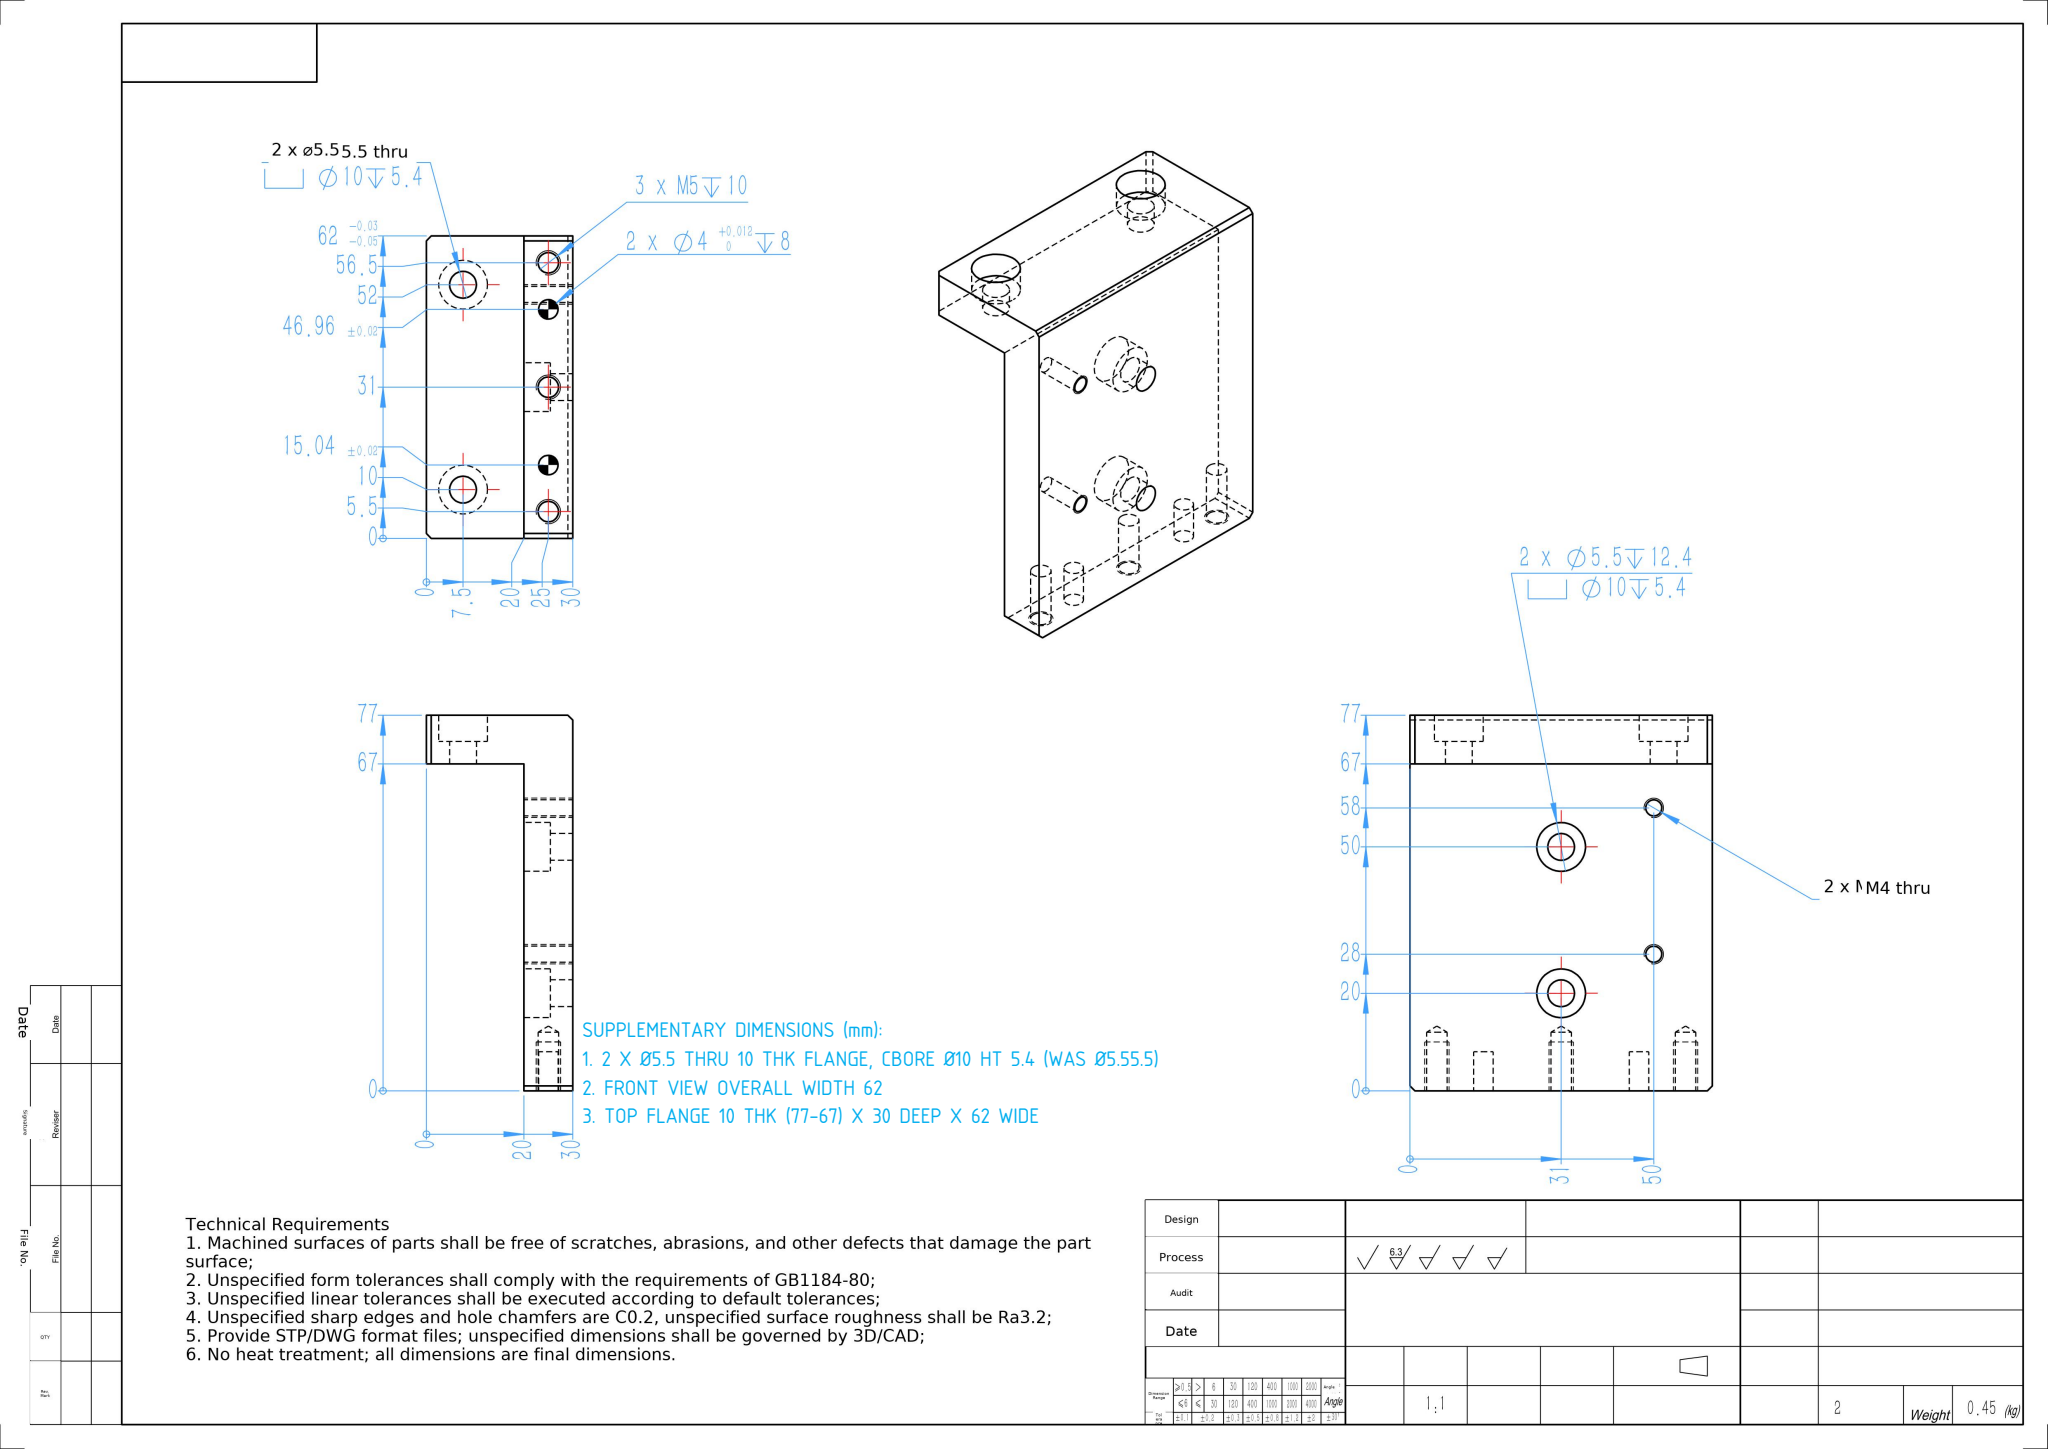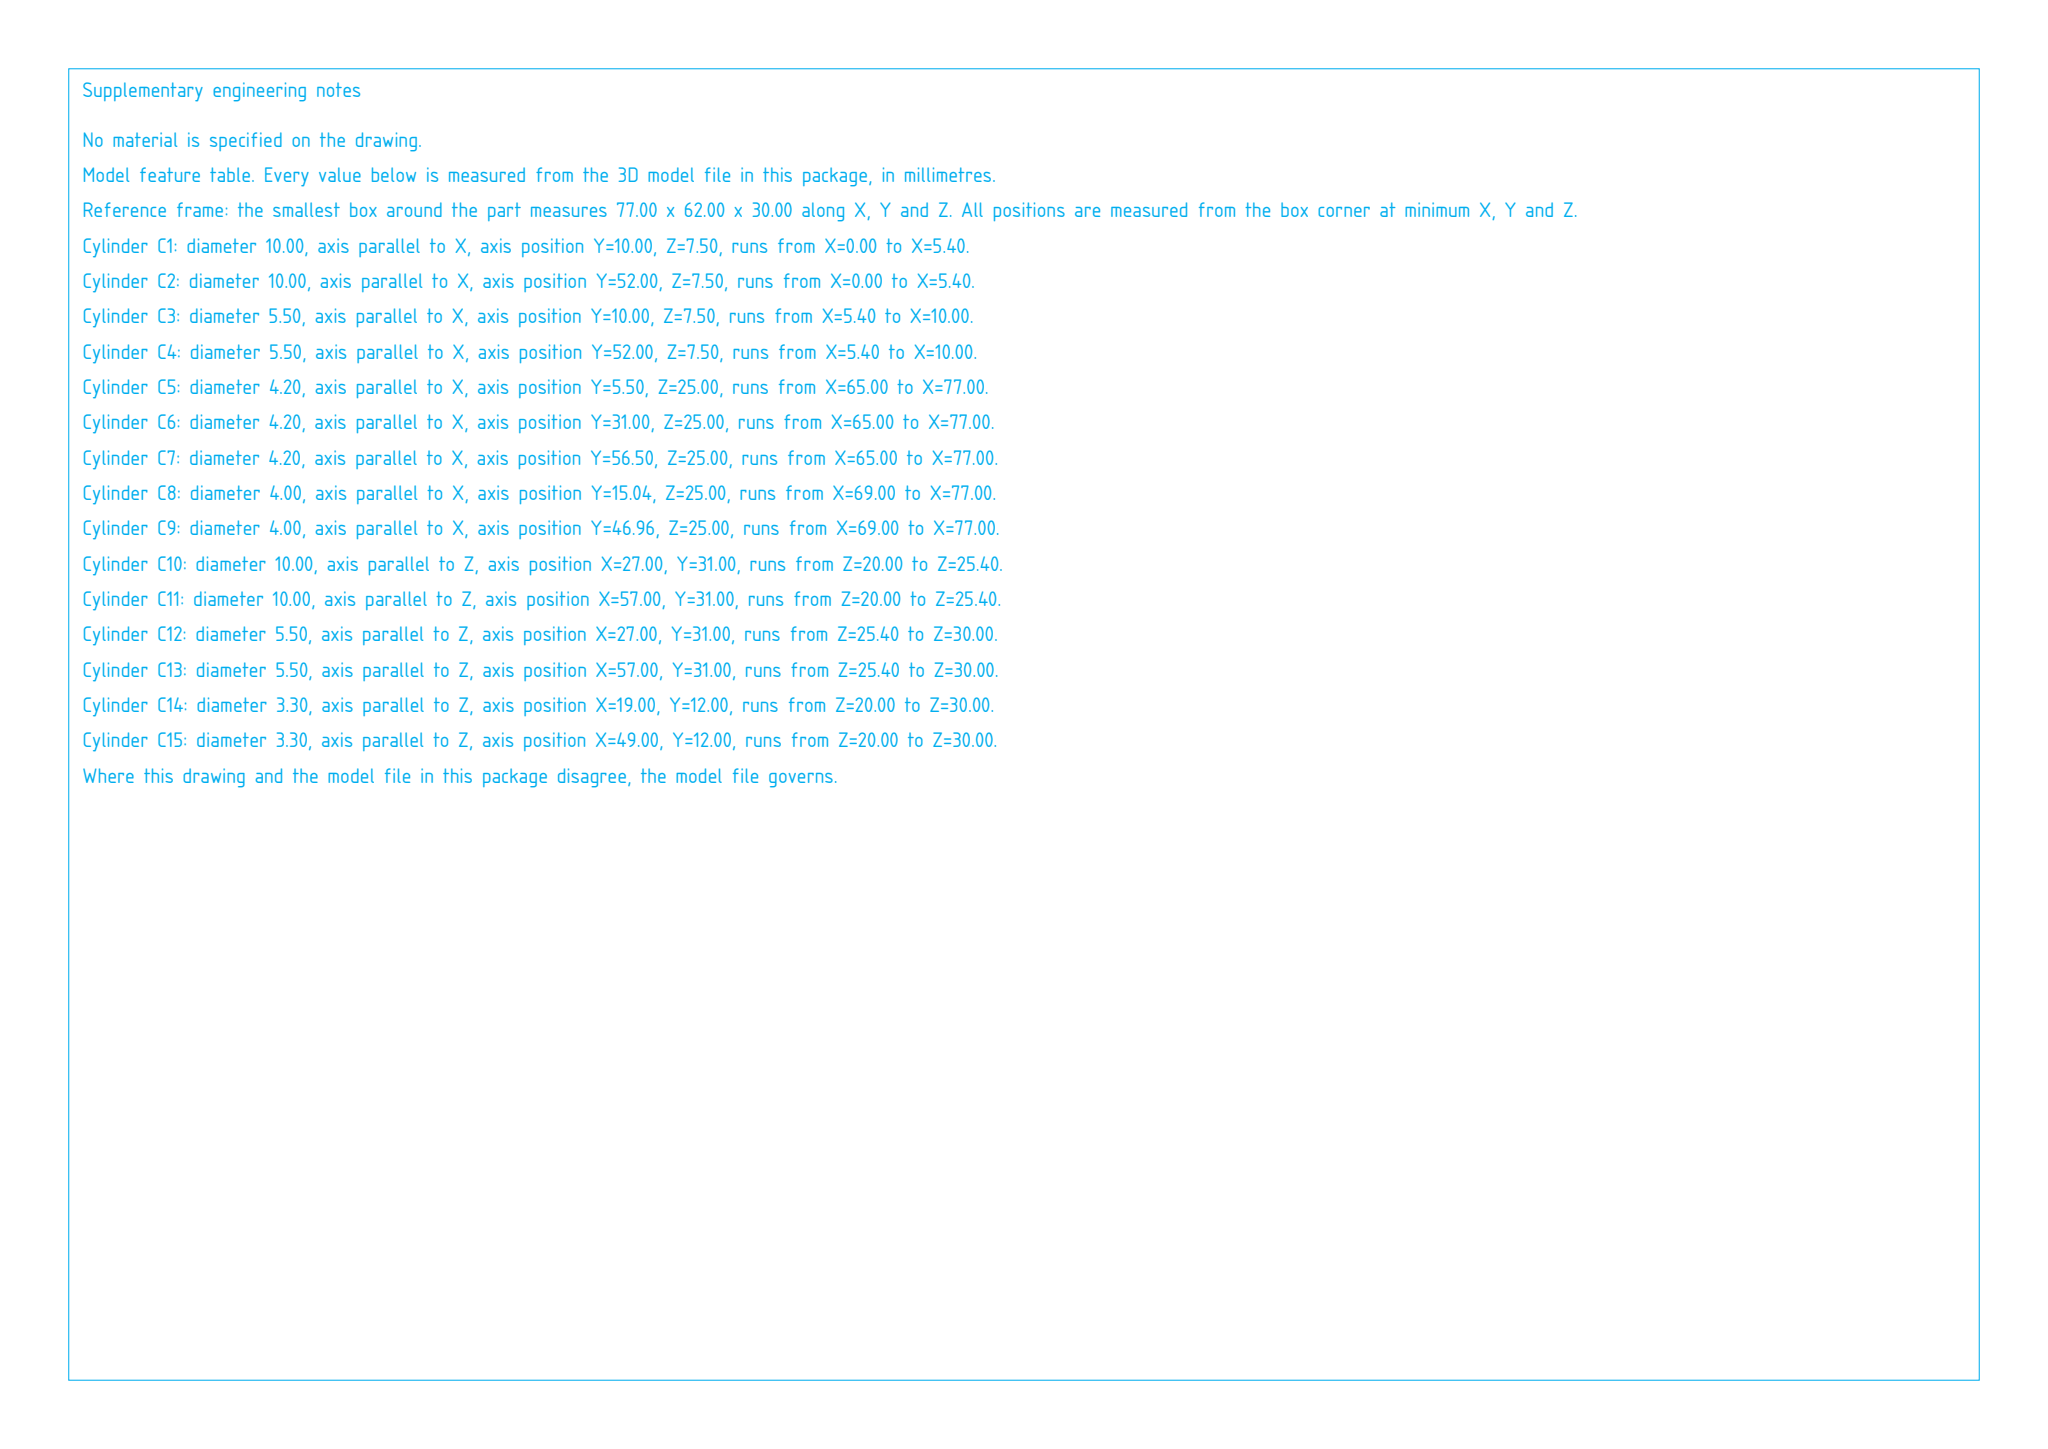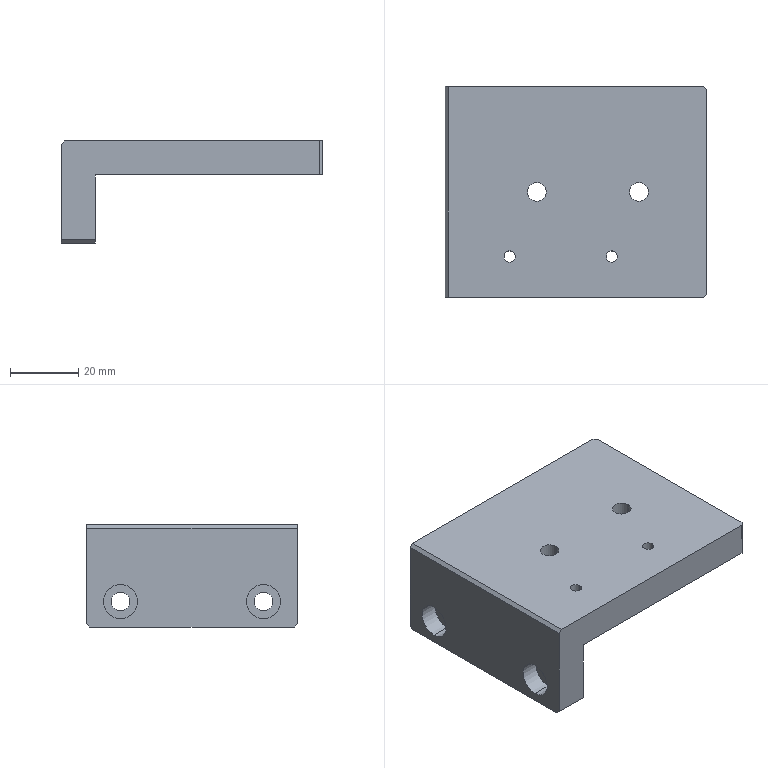Part | SolidWorks | mm | 1 solid | 55 faces | box 77 x 62 x 30 mm | volume 57067 mm3 | cylinder 30 | plane 19 | cone 6 | commonest cylinder face diameters 10 x8 5.5 x8 4.2 x6 3.3 x4 4 x4
build123d program:
from build123d import *

# Parameters (mm, degrees)
SKETCH1_W                                       = 77
SKETCH1_H                                       = 62
BOSS_EXTRUDE1_DEPTH                             = 30
SKETCH2_W                                       = 67
SKETCH2_H                                       = 20
CUT_EXTRUDE1_DEPTH                              = 79.907
CHAMFER1_SIZE                                   = 1
M5_HEX_SOCKET_HEAD_CAP_SCREW_CBORE1_D           = 5.5
M5_HEX_SOCKET_HEAD_CAP_SCREW_CBORE1_CBORE_D     = 10
M5_HEX_SOCKET_HEAD_CAP_SCREW_CBORE1_CBORE_DEPTH = 5.4
M5_HEX_SOCKET_HEAD_CAP_SCREW_CBORE2_D           = 5.5
M5_HEX_SOCKET_HEAD_CAP_SCREW_CBORE2_DEPTH       = 12.4
M5_HEX_SOCKET_HEAD_CAP_SCREW_CBORE2_CBORE_D     = 10
M5_HEX_SOCKET_HEAD_CAP_SCREW_CBORE2_CBORE_DEPTH = 5.4
M5_HEX_SOCKET_HEAD_CAP_SCREW_CBORE2_TIP         = 1.652
M5_TAPPED_HOLE1_D                               = 4.2
M5_TAPPED_HOLE1_DEPTH                           = 12
M5_TAPPED_HOLE1_TIP                             = 1.262
F_4_0MM_DOWEL_HOLE_1_D                          = 4
F_4_0MM_DOWEL_HOLE_1_DEPTH                      = 8
M4_TAPPED_HOLE1_D                               = 3.3


with BuildPart() as part:
    # Sketch1 → Boss-Extrude1 (new body)
    with BuildSketch(Plane.XY):
        Rectangle(SKETCH1_W, SKETCH1_H)
    extrude(amount=BOSS_EXTRUDE1_DEPTH)

    # Sketch2 → Cut-Extrude1 (cut, through all)
    with BuildSketch(Plane(origin=(0, 31, 0), x_dir=(1, 0, 0), z_dir=(0, 1, 0))):
        with Locations((5, -10)):
            Rectangle(SKETCH2_W, SKETCH2_H)
    extrude(amount=-CUT_EXTRUDE1_DEPTH, mode=Mode.SUBTRACT)

    # Chamfer1
    chamfer1_edges = [part.edges().sort_by_distance(p)[0] for p in [
        (-38.5, 0, 30),
        (-33.5, 31, 0),
        (-33.5, -31, 0),
        (38.5, -31, 25),
        (38.5, 31, 25),
    ]]
    chamfer(chamfer1_edges, length=CHAMFER1_SIZE)

    # M5 Hex Socket Head Cap Screw CBORE1 (through all)
    with Locations(Plane.ZY.offset(38.5)):
        with Locations((7.5, 21), (7.5, -21)):
            CounterBoreHole(M5_HEX_SOCKET_HEAD_CAP_SCREW_CBORE1_D / 2, M5_HEX_SOCKET_HEAD_CAP_SCREW_CBORE1_CBORE_D / 2, M5_HEX_SOCKET_HEAD_CAP_SCREW_CBORE1_CBORE_DEPTH)

    # M5 Hex Socket Head Cap Screw CBORE2
    with Locations(Plane(origin=(0, 0, 20), x_dir=(-1, 0, 0), z_dir=(0, 0, -1))):
        with Locations((11.5, 0), (-18.5, 0)):
            CounterBoreHole(M5_HEX_SOCKET_HEAD_CAP_SCREW_CBORE2_D / 2, M5_HEX_SOCKET_HEAD_CAP_SCREW_CBORE2_CBORE_D / 2, M5_HEX_SOCKET_HEAD_CAP_SCREW_CBORE2_CBORE_DEPTH, depth=M5_HEX_SOCKET_HEAD_CAP_SCREW_CBORE2_DEPTH)
            with Locations((0, 0, -(M5_HEX_SOCKET_HEAD_CAP_SCREW_CBORE2_DEPTH + M5_HEX_SOCKET_HEAD_CAP_SCREW_CBORE2_TIP / 2))):  # 118° drill point
                Cone(0, M5_HEX_SOCKET_HEAD_CAP_SCREW_CBORE2_D / 2, M5_HEX_SOCKET_HEAD_CAP_SCREW_CBORE2_TIP, mode=Mode.SUBTRACT)

    # M5 Tapped Hole1
    with Locations(Plane(origin=(38.5, 0, 0), x_dir=(0, 0, -1), z_dir=(1, 0, 0))):
        with Locations((-25, -25.5), (-25, 25.5), (-25, 0)):
            Hole(M5_TAPPED_HOLE1_D / 2, depth=M5_TAPPED_HOLE1_DEPTH)
            with Locations((0, 0, -(M5_TAPPED_HOLE1_DEPTH + M5_TAPPED_HOLE1_TIP / 2))):  # 118° drill point
                Cone(0, M5_TAPPED_HOLE1_D / 2, M5_TAPPED_HOLE1_TIP, mode=Mode.SUBTRACT)

    # 4.0mm Dowel Hole 1
    with Locations(Plane(origin=(38.5, 0, 0), x_dir=(0, 0, -1), z_dir=(1, 0, 0))):
        with Locations((-25, -15.958), (-25, 15.958)):
            Hole(F_4_0MM_DOWEL_HOLE_1_D / 2, depth=F_4_0MM_DOWEL_HOLE_1_DEPTH)

    # M4 Tapped Hole1 (through all)
    with Locations(Plane.XY.offset(30)):
        with Locations((-19.5, -19), (10.5, -19)):
            Hole(M4_TAPPED_HOLE1_D / 2)


solid = part.part